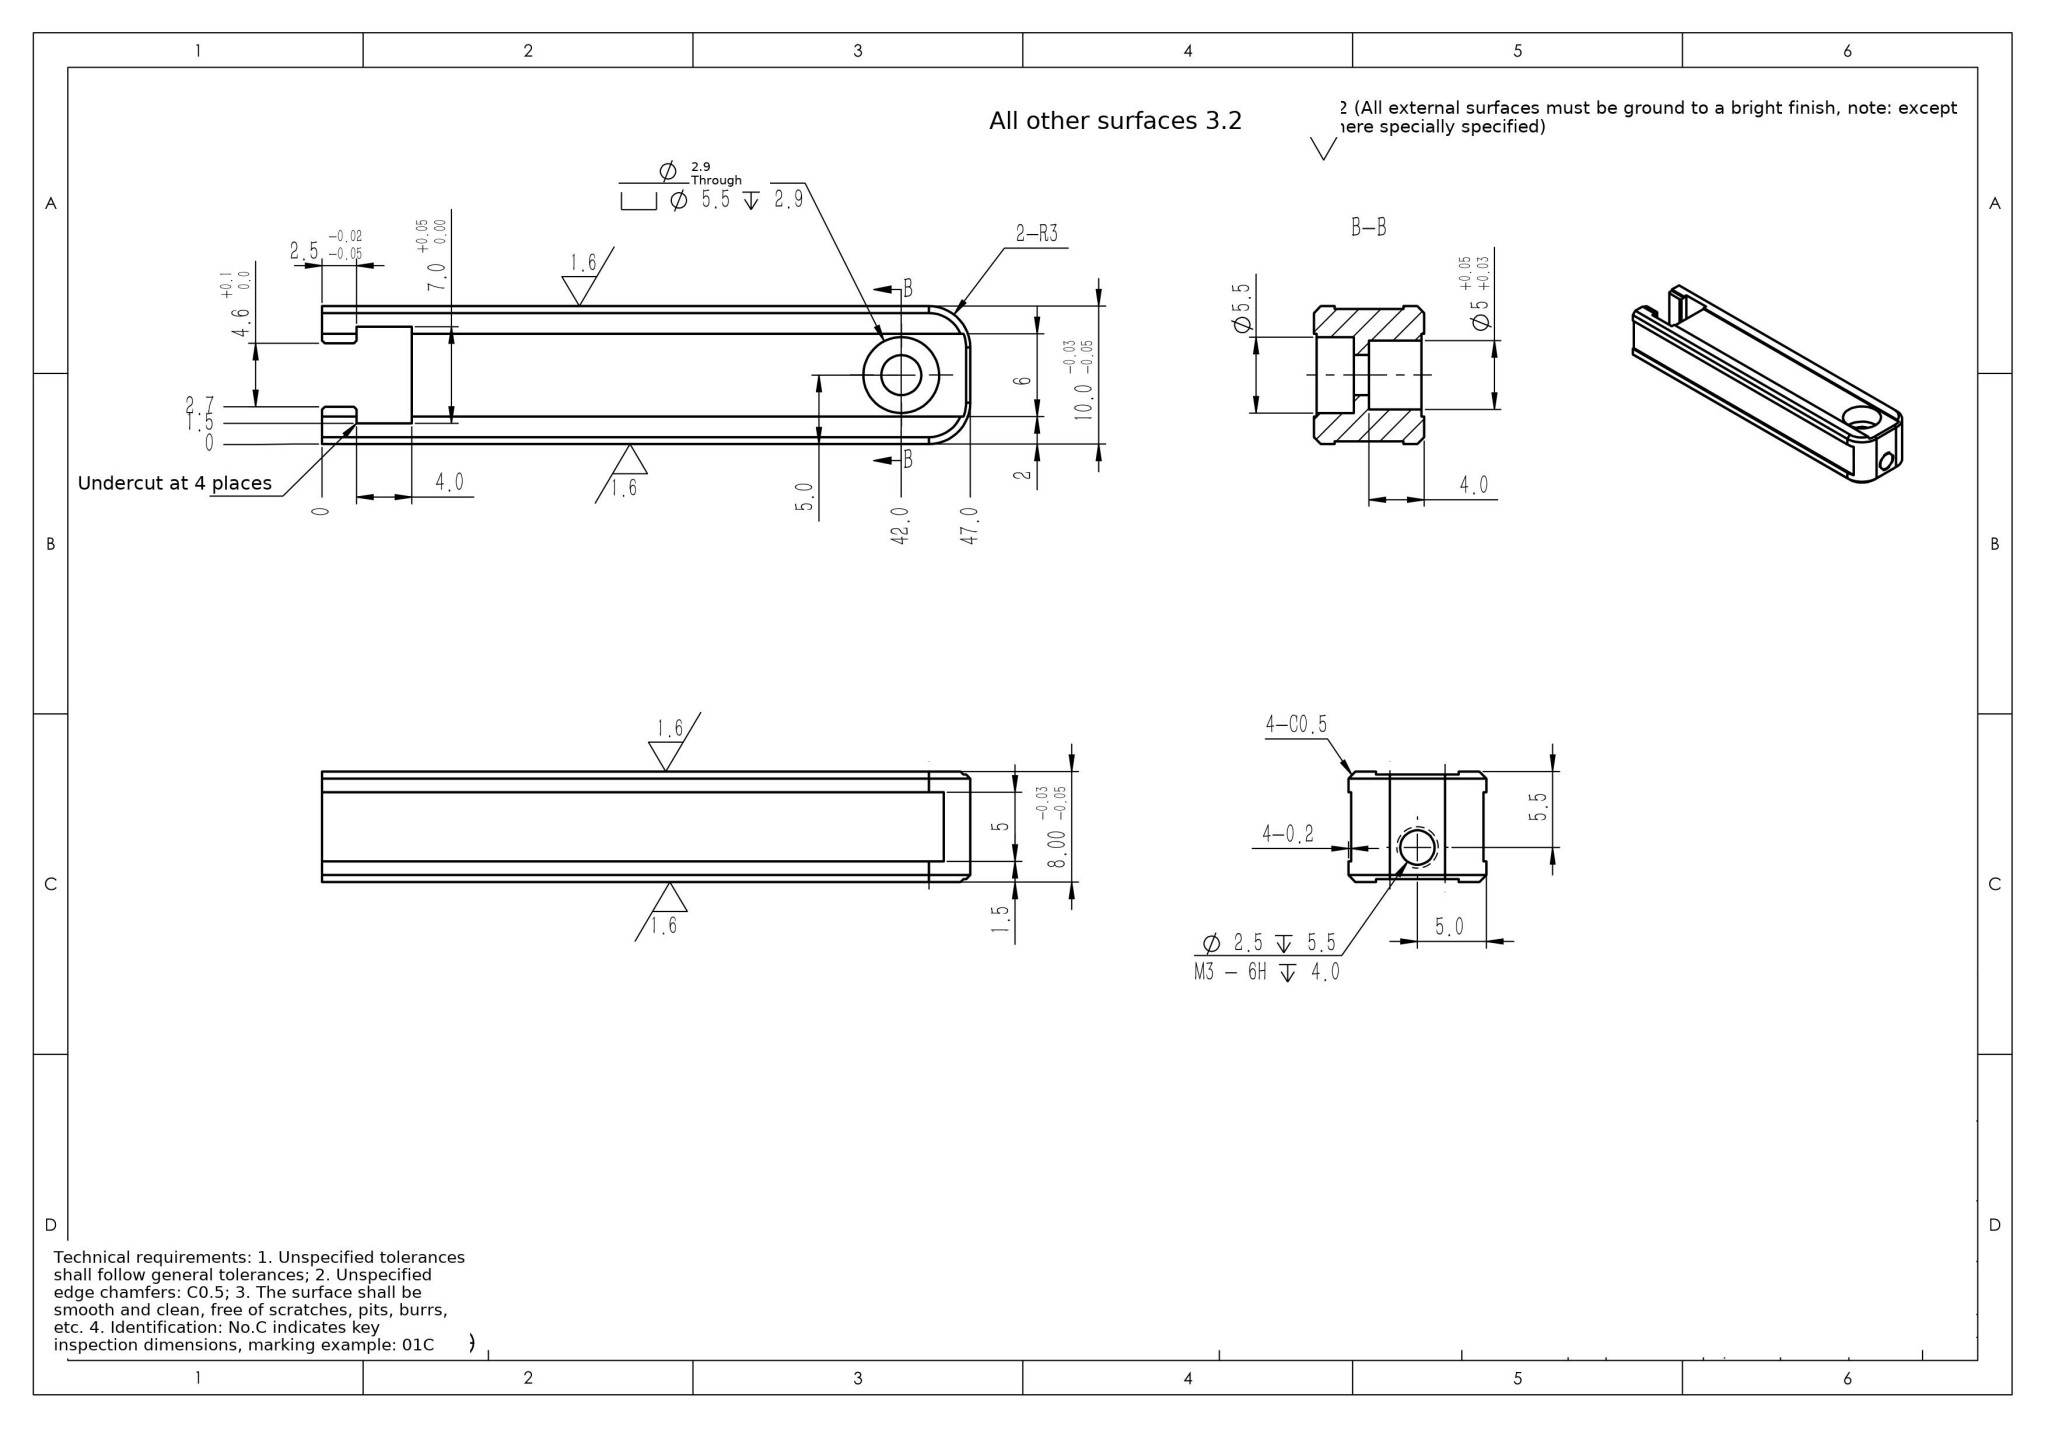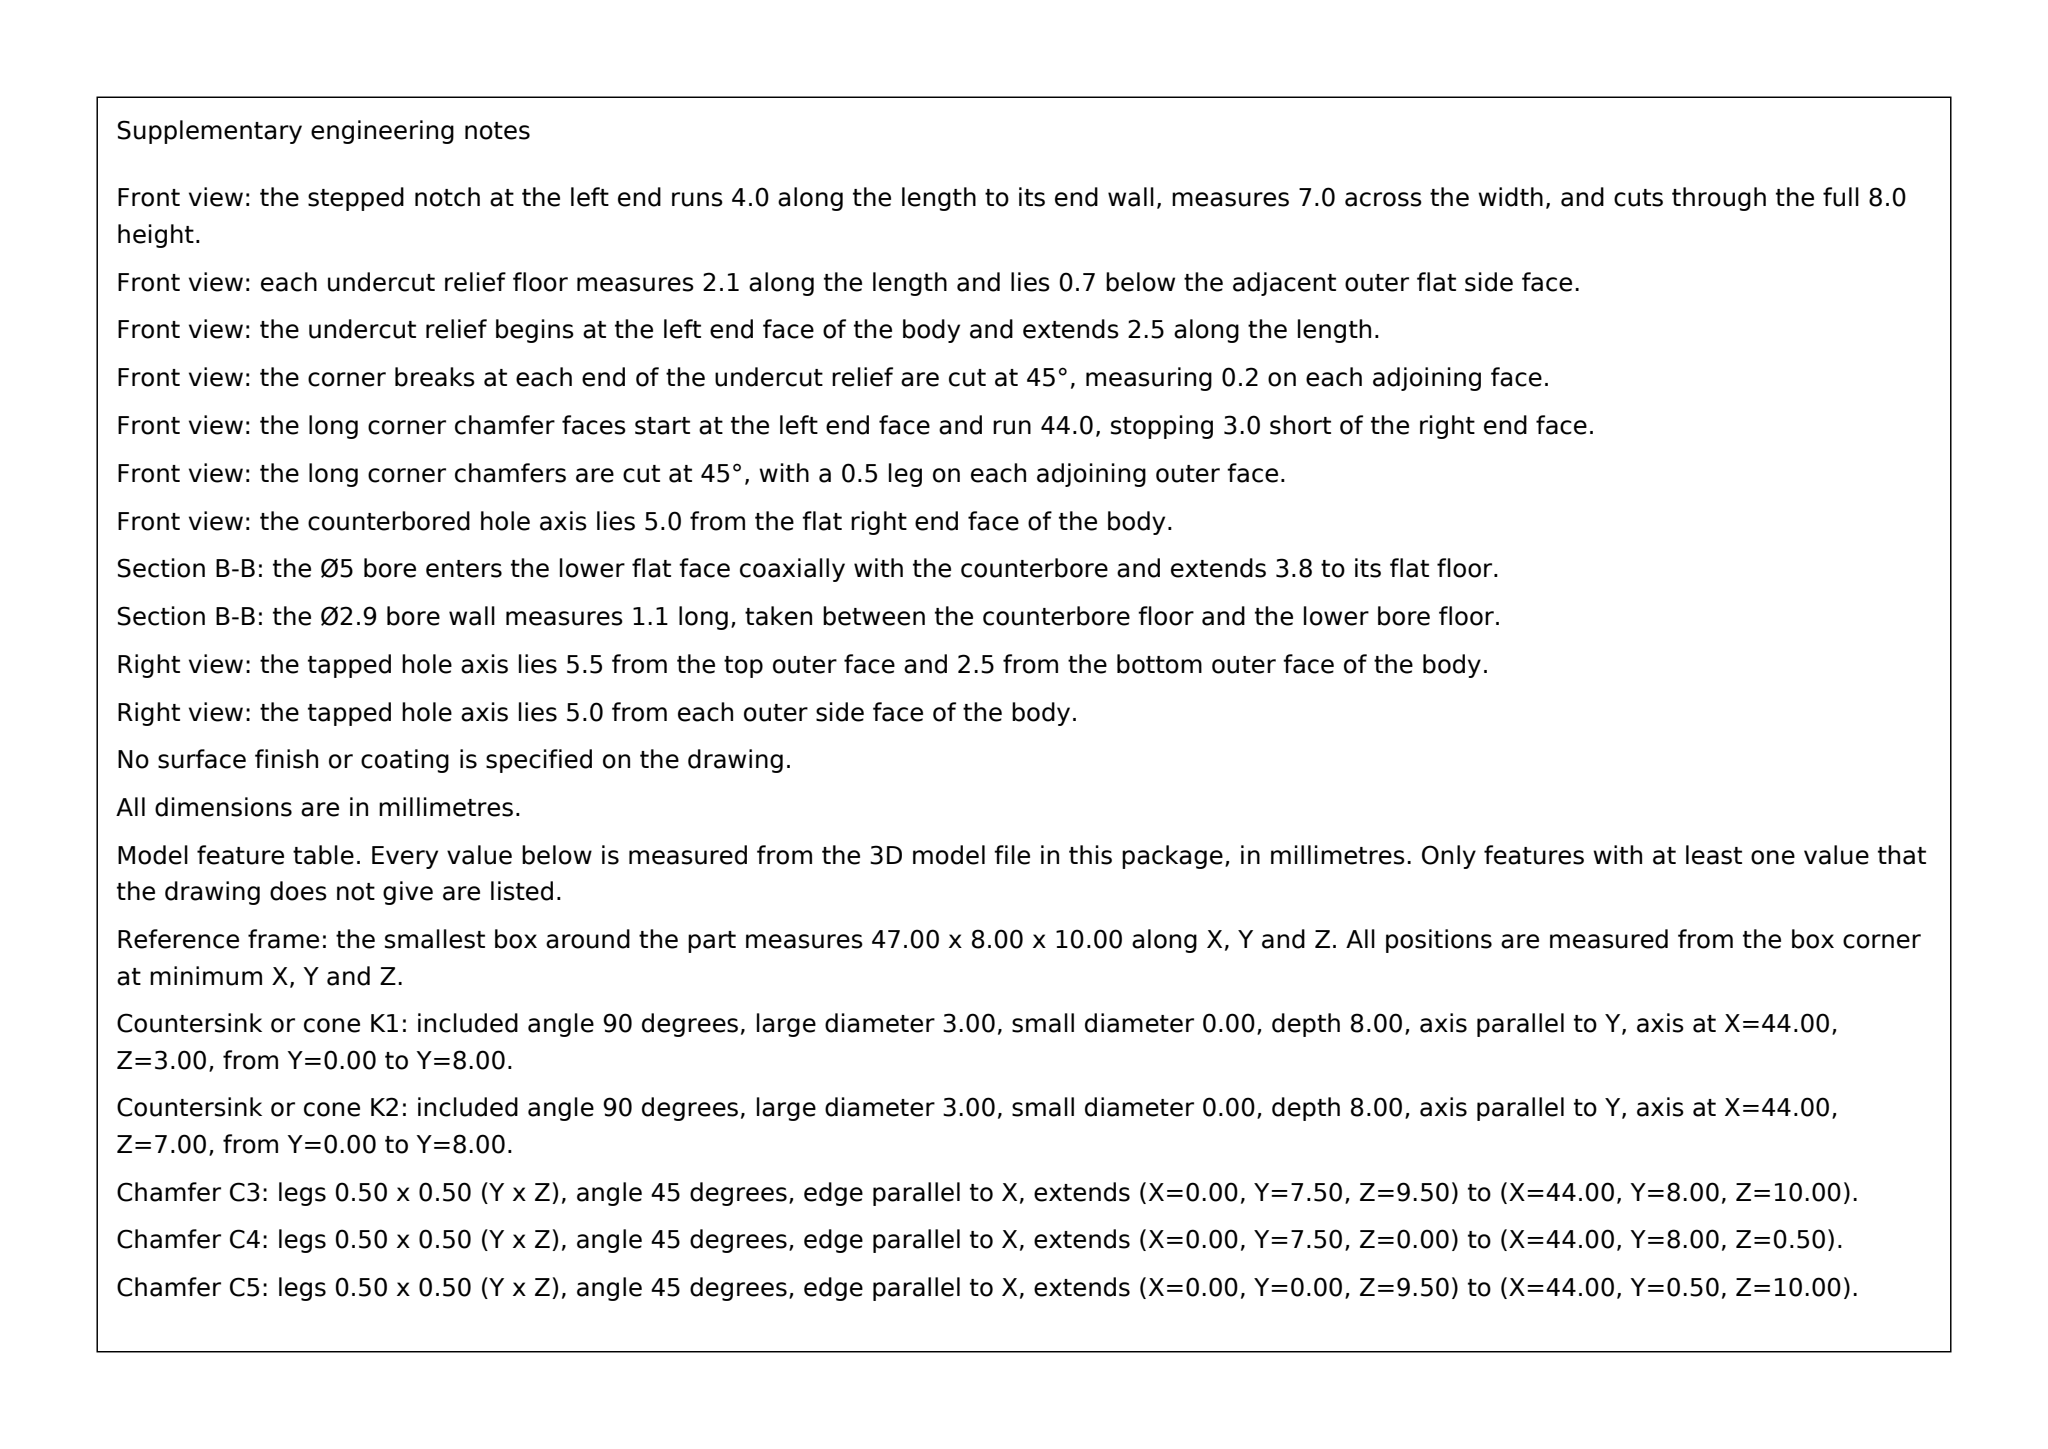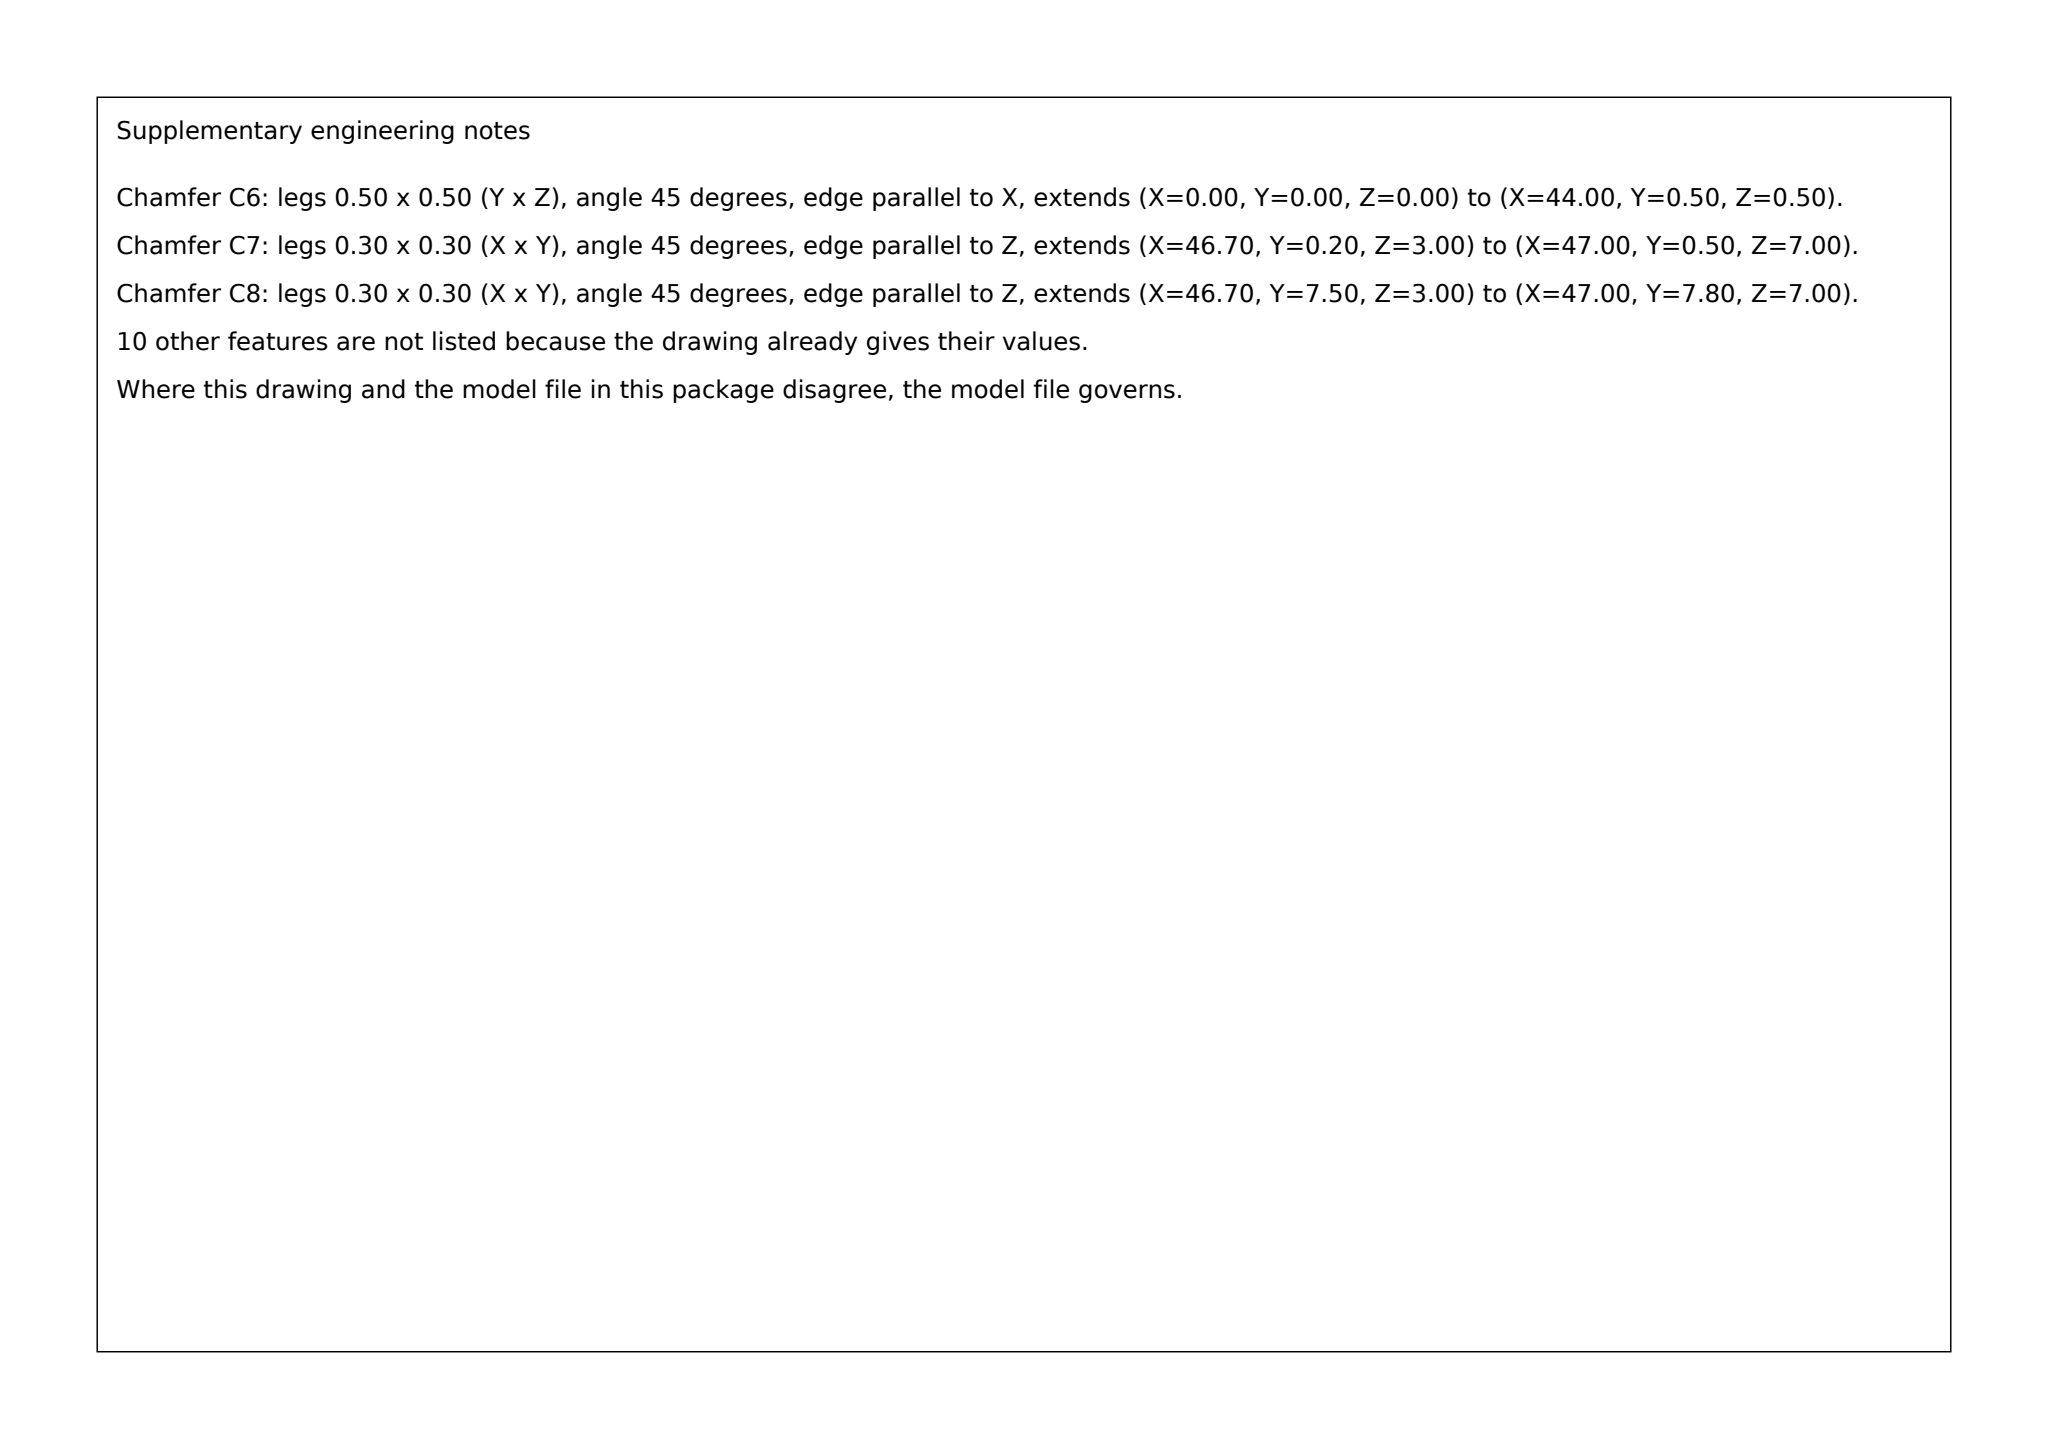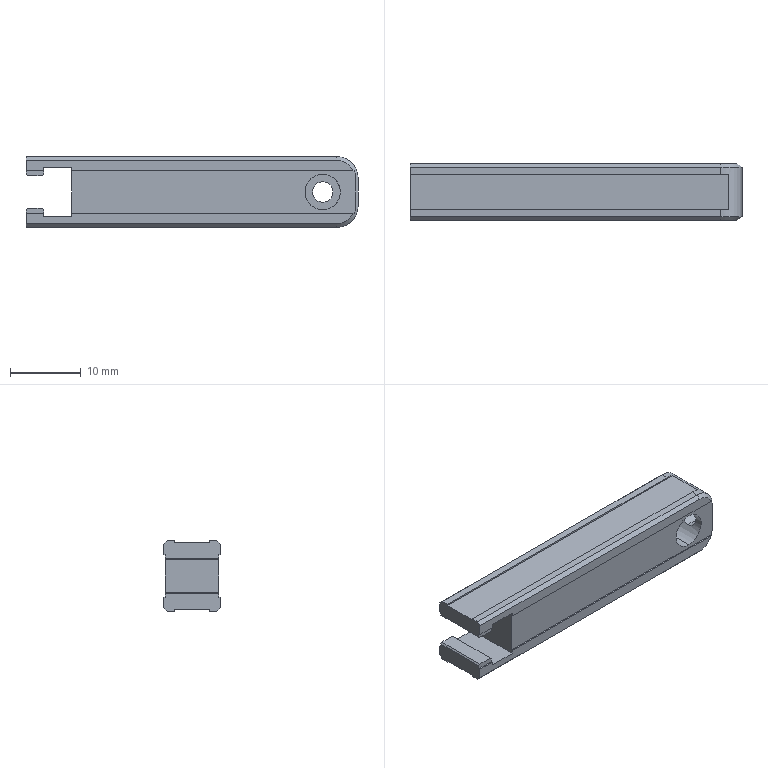Part | SolidWorks | mm | 1 solid | 64 faces | box 47 x 8 x 10 mm | volume 3042 mm3 | plane 50 | cylinder 10 | cone 4 | commonest cylinder face diameters 2.5 x2 2.9 x2 5.5 x2 5 x2 6 x2
Drawing notes:
OPEN SLOT 6.0 WIDE x 6.5 DP FROM LEFT END FACE | from the solid: z-planes 2.0 & 8.0 give 6.0 slot width; x-plane 6.5 slot bottom vs x=0 end face = 6.5 DP (2.5 undercut + 4.0)
M3-6H TAP DP 4.0 ON Ø2.5 DRILL DP 5.5, axis parallel to the 47.0 length (hole normal to an end face); hole centre located 2.5 from the Y=0 side face and 5.0 from the Z=0 bottom face. | from the solid: cylinders[dia,axis,pos_other_axes,length]: [2.5,"x",[null,2.5,5.0],2.83]
Ø5 +0.05/+0.03 bore (callout to be added on the main view): axis normal to the 47.0 x 10.0 face, located 42.0 from the left end face and 5.0 from the bottom face; bore axial extent 3.8, coaxial with Ø5.5 (extent 2.7) and Ø2.9 THRU (extent 1.1). | from the solid: cylinders: [5.0,"y",[42.0,null,5.0],3.8]; [5.5,"y",[42.0,null,5.0],2.7]; [2.9,"y",[42.0,null,5.0],1.1]
Left-end open slot: 6.0 wide x 6.5 deep measured from the X=0 end face (slot bottom face at X=6.5 from the left end face). | from the solid: axis_planes: ["x",6.5,1] with ["x",0.0,2]
Longitudinal top channel cross-section: 5.0 wide between faces at Y=1.5 and Y=6.5 from the Y=0 side face, floor at Y=4.0 (depth 4.0 from the Y=8.0 face). | from the solid: axis_planes: ["y",1.5,2], ["y",6.5,2], ["y",4.0,1], ["y",8.0,2]
build123d program:
from build123d import *

# Parameters (mm, degrees)
SKETCH1_W                                         = 47
SKETCH1_H                                         = 10
BOSS_EXTRUDE1_DEPTH                               = 8
SKETCH4_W                                         = 13
SKETCH4_H                                         = 4.6
CUT_EXTRUDE1_DEPTH                                = 26.323
SKETCH5_W                                         = 4
SKETCH5_H                                         = 7
CUT_EXTRUDE2_DEPTH                                = 26.323
FILLET1_R                                         = 3
SKETCH9_R                                         = 2.5
CUT_EXTRUDE3_DEPTH                                = 4
M2_5_HEX_SOCKET_HEAD_CAP_SCREW_CBORE1_D           = 2.9
M2_5_HEX_SOCKET_HEAD_CAP_SCREW_CBORE1_DEPTH       = 8.5
M2_5_HEX_SOCKET_HEAD_CAP_SCREW_CBORE1_CBORE_D     = 5.5
M2_5_HEX_SOCKET_HEAD_CAP_SCREW_CBORE1_CBORE_DEPTH = 2.9
M2_5_HEX_SOCKET_HEAD_CAP_SCREW_CBORE1_TIP         = 0.8712
CHAMFER1_SIZE                                     = 0.5
M3_TAPPED_HOLE1_D                                 = 2.5
M3_TAPPED_HOLE1_DEPTH                             = 5.5
M3_TAPPED_HOLE1_TIP                               = 0.7511
CHAMFER2_SIZE                                     = 0.2
SKETCH14_W                                        = 47
SKETCH14_H                                        = 5
CUT_EXTRUDE4_DEPTH                                = 0.2
SKETCH15_W                                        = 47
SKETCH15_H                                        = 5
CUT_EXTRUDE5_DEPTH                                = 0.2
SKETCH16_W                                        = 47
SKETCH16_H                                        = 6
CUT_EXTRUDE6_DEPTH                                = 0.2
SKETCH17_W                                        = 47
SKETCH17_H                                        = 6
CUT_EXTRUDE7_DEPTH                                = 0.2


with BuildPart() as part:
    # Sketch1 → Boss-Extrude1 (new body)
    with BuildSketch(Plane(origin=(0, 0, 0), x_dir=(1, 0, 0), z_dir=(0, 1, 0))):
        Rectangle(SKETCH1_W, SKETCH1_H)
    extrude(amount=BOSS_EXTRUDE1_DEPTH)

    # Sketch4 → Cut-Extrude1 (cut, through all)
    with BuildSketch(Plane.XZ):
        with Locations((-23.5, 0)):
            Rectangle(SKETCH4_W, SKETCH4_H)
    extrude(amount=-CUT_EXTRUDE1_DEPTH, mode=Mode.SUBTRACT)

    # Sketch5 → Cut-Extrude2 (cut, through all)
    with BuildSketch(Plane.XZ):
        with Locations((-19, 0)):
            Rectangle(SKETCH5_W, SKETCH5_H)
    extrude(amount=-CUT_EXTRUDE2_DEPTH, mode=Mode.SUBTRACT)

    # Fillet1
    fillet1_edges = [part.edges().sort_by_distance(p)[0] for p in [
        (23.5, 4, 5),
        (23.5, 4, -5),
    ]]
    fillet(fillet1_edges, radius=FILLET1_R)

    # Sketch9 → Cut-Extrude3 (cut)
    with BuildSketch(Plane.XZ):
        with Locations(Location((18.5, 0, 0), (0, 0, 270))):
            Circle(SKETCH9_R)
    extrude(amount=-CUT_EXTRUDE3_DEPTH, mode=Mode.SUBTRACT)

    # M2.5 Hex Socket Head Cap Screw CBORE1
    with Locations(Plane(origin=(0, 8, 0), x_dir=(1, 0, 0), z_dir=(0, 1, 0))):
        with Locations((18.5, 0)):
            CounterBoreHole(M2_5_HEX_SOCKET_HEAD_CAP_SCREW_CBORE1_D / 2, M2_5_HEX_SOCKET_HEAD_CAP_SCREW_CBORE1_CBORE_D / 2, M2_5_HEX_SOCKET_HEAD_CAP_SCREW_CBORE1_CBORE_DEPTH, depth=M2_5_HEX_SOCKET_HEAD_CAP_SCREW_CBORE1_DEPTH)
            with Locations((0, 0, -(M2_5_HEX_SOCKET_HEAD_CAP_SCREW_CBORE1_DEPTH + M2_5_HEX_SOCKET_HEAD_CAP_SCREW_CBORE1_TIP / 2))):  # 118° drill point
                Cone(0, M2_5_HEX_SOCKET_HEAD_CAP_SCREW_CBORE1_D / 2, M2_5_HEX_SOCKET_HEAD_CAP_SCREW_CBORE1_TIP, mode=Mode.SUBTRACT)

    # Chamfer1
    chamfer1_edges = [part.edges().sort_by_distance(p)[0] for p in [
        (-1.5, 8, 5),
        (-1.5, 0, 5),
        (23.5, 0, 0),
        (23.5, 8, 0),
        (-1.5, 0, -5),
        (22.621, 0, -4.121),
        (22.621, 0, 4.121),
        (-1.5, 8, -5),
        (22.621, 8, -4.121),
        (22.621, 8, 4.121),
    ]]
    chamfer(chamfer1_edges, length=CHAMFER1_SIZE)

    # M3 Tapped Hole1
    with Locations(Plane(origin=(23.5, 0, 0), x_dir=(0, 0, -1), z_dir=(1, 0, 0))):
        with Locations((0, 2.5)):
            Hole(M3_TAPPED_HOLE1_D / 2, depth=M3_TAPPED_HOLE1_DEPTH)
            with Locations((0, 0, -(M3_TAPPED_HOLE1_DEPTH + M3_TAPPED_HOLE1_TIP / 2))):  # 118° drill point
                Cone(0, M3_TAPPED_HOLE1_D / 2, M3_TAPPED_HOLE1_TIP, mode=Mode.SUBTRACT)

    # Chamfer2
    chamfer2_edges = [part.edges().sort_by_distance(p)[0] for p in [
        (-23.5, 4, -2.3),
        (-23.5, 4, 2.3),
        (-21, 4, 2.3),
        (-21, 4, -2.3),
    ]]
    chamfer(chamfer2_edges, length=CHAMFER2_SIZE)

    # Sketch14 → Cut-Extrude4 (cut)
    with BuildSketch(Plane(origin=(0, 0, -5), x_dir=(-1, 0, 0), z_dir=(0, 0, -1))):
        with Locations((0, 4)):
            Rectangle(SKETCH14_W, SKETCH14_H)
    extrude(amount=-CUT_EXTRUDE4_DEPTH, mode=Mode.SUBTRACT)

    # Sketch15 → Cut-Extrude5 (cut)
    with BuildSketch(Plane.XY.offset(5)):
        with Locations((0, 4)):
            Rectangle(SKETCH15_W, SKETCH15_H)
    extrude(amount=-CUT_EXTRUDE5_DEPTH, mode=Mode.SUBTRACT)

    # Sketch16 → Cut-Extrude6 (cut)
    with BuildSketch(Plane(origin=(0, 8, 0), x_dir=(1, 0, 0), z_dir=(0, 1, 0))):
        Rectangle(SKETCH16_W, SKETCH16_H)
    extrude(amount=-CUT_EXTRUDE6_DEPTH, mode=Mode.SUBTRACT)

    # Sketch17 → Cut-Extrude7 (cut)
    with BuildSketch(Plane.XZ):
        Rectangle(SKETCH17_W, SKETCH17_H)
    extrude(amount=-CUT_EXTRUDE7_DEPTH, mode=Mode.SUBTRACT)


solid = part.part